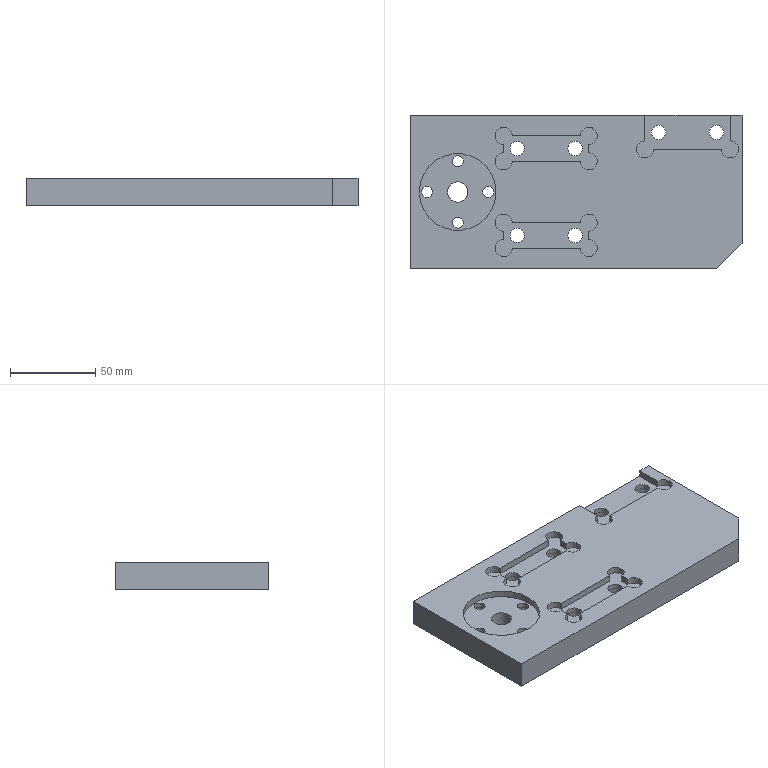Component | NX | BASE_PLATE | 1 solid | 64 faces | volume 245771 mm3 | cylinder 32 | plane 32 | commonest cylinder face diameters 10 x10 8.5 x6 14 x6 6.5 x4 11 x4 12 x1 45 x1